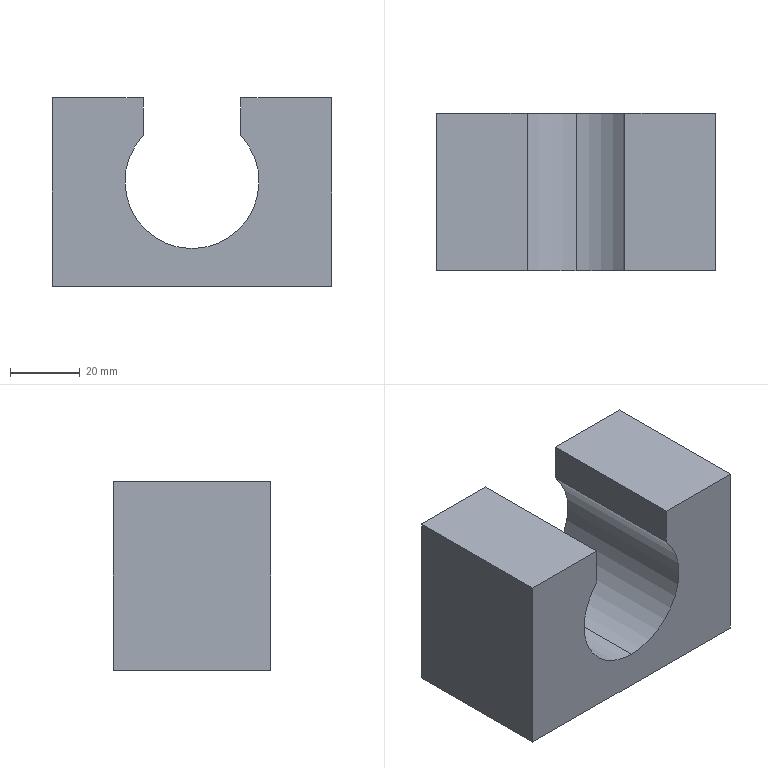Component | SolidWorks | 30-24A-1 | 1 solid | 43 faces | box 80 x 45 x 54 mm | volume 129747 mm3 | cylinder 18 | cone 16 | plane 9 | commonest cylinder face diameters 4.2 x8 6.8 x8 38.4 x2
build123d program:
from build123d import *

# Parameters (mm, degrees)
EXTRUDE1_DEPTH        = 22.5
M8_TAPPED_HOLE1_D     = 6.8
M8_TAPPED_HOLE1_DEPTH = 22.25
M8_TAPPED_HOLE1_TIP   = 2.043
M5_TAPPED_HOLE1_D     = 4.2
M5_TAPPED_HOLE1_DEPTH = 14
M5_TAPPED_HOLE1_TIP   = 1.262


with BuildPart() as part:
    # Sketch4 → Extrude1 (new, symmetric)
    with BuildSketch(Plane(origin=(0, 0, 0), x_dir=(1, 0, 0), z_dir=(0, 1, 0))):
        with BuildLine():
            Line((-40, 27), (40, 27))
            Line((40, 27), (40, -27))
            Line((40, -27), (14, -27))
            Line((14, -27), (14, -16.139))
            ThreePointArc((14, -16.139), (0, 16.2), (-14, -16.139))
            Line((-14, -16.139), (-14, -27))
            Line((-14, -27), (-40, -27))
            Line((-40, -27), (-40, 27))
        make_face()
    extrude(amount=EXTRUDE1_DEPTH, both=True)

    # M8 Tapped Hole1
    with Locations(Plane(origin=(48.016, 4.273, -27), x_dir=(-1, 0, 0), z_dir=(0, 0, -1))):
        with Locations((15.516, 10.727), (15.516, -19.273), (80.516, -19.273), (80.516, 10.727)):
            Hole(M8_TAPPED_HOLE1_D / 2, depth=M8_TAPPED_HOLE1_DEPTH)
            with Locations((0, 0, -(M8_TAPPED_HOLE1_DEPTH + M8_TAPPED_HOLE1_TIP / 2))):  # 118° drill point
                Cone(0, M8_TAPPED_HOLE1_D / 2, M8_TAPPED_HOLE1_TIP, mode=Mode.SUBTRACT)

    # M5 Tapped Hole1
    with Locations(Plane.XZ.offset(22.5)):
        with Locations((21.651, -9.5), (21.651, 15.5), (-21.651, 15.5), (-21.651, -9.5)):
            Hole(M5_TAPPED_HOLE1_D / 2, depth=M5_TAPPED_HOLE1_DEPTH)
            with Locations((0, 0, -(M5_TAPPED_HOLE1_DEPTH + M5_TAPPED_HOLE1_TIP / 2))):  # 118° drill point
                Cone(0, M5_TAPPED_HOLE1_D / 2, M5_TAPPED_HOLE1_TIP, mode=Mode.SUBTRACT)


solid = part.part

# Placed as in the assembly
solid = solid.moved(Location((-649.208, -37.092, 66.188), (0, 0, 180)))